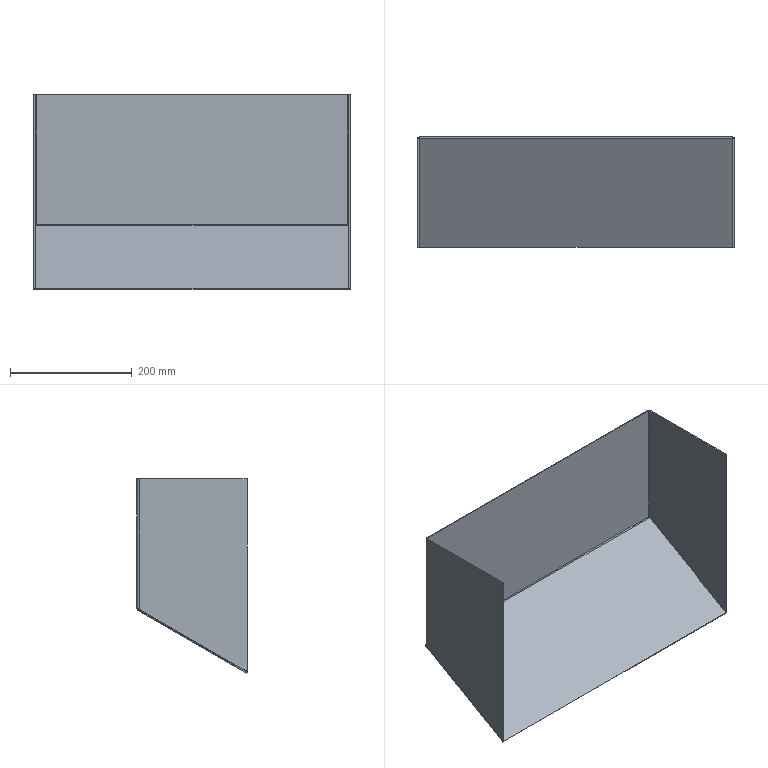Component | SolidWorks | RearLeftSidePlateAssembly-2_RearLeftSidePlateAirInletBaffle-3 | 1 solid | 32 faces | box 520 x 181 x 320 mm | volume 628304 mm3 | plane 24 | cylinder 6 | spline 2 | commonest cylinder face diameters 8 x3 4 x3 | material Plain Carbon Steel
STEP:
#1=COLOUR_RGB('',0.7922,0.8196,0.9333);
#2=FILL_AREA_STYLE_COLOUR('',#1);
#3=FILL_AREA_STYLE('',(#2));
#4=SURFACE_STYLE_FILL_AREA(#3);
#5=SURFACE_SIDE_STYLE('',(#4));
#6=SURFACE_STYLE_USAGE(.BOTH.,#5);
#7=PRESENTATION_STYLE_ASSIGNMENT((#6));
#8=CARTESIAN_POINT('',(98.555,5.691,77.381));
#9=VERTEX_POINT('',#8);
#10=CARTESIAN_POINT('',(98.555,5.691,68.965));
#11=VERTEX_POINT('',#10);
#12=CARTESIAN_POINT('',(98.555,5.691,77.381));
#13=DIRECTION('',(0.,-0.,-1.));
#14=VECTOR('',#13,39.37);
#15=LINE('',#12,#14);
#16=EDGE_CURVE('',#9,#11,#15,.T.);
#17=ORIENTED_EDGE('',*,*,#16,.F.);
#18=CARTESIAN_POINT('',(78.397,5.691,77.381));
#19=VERTEX_POINT('',#18);
#20=CARTESIAN_POINT('',(78.24,5.691,77.381));
#21=DIRECTION('',(1.,0.,-0.));
#22=VECTOR('',#21,39.37);
#23=LINE('',#20,#22);
#24=EDGE_CURVE('',#19,#9,#23,.T.);
#25=ORIENTED_EDGE('',*,*,#24,.F.);
#26=CARTESIAN_POINT('',(78.397,5.691,68.965));
#27=VERTEX_POINT('',#26);
#28=CARTESIAN_POINT('',(78.397,5.691,68.92));
#29=DIRECTION('',(-0.,0.,1.));
#30=VECTOR('',#29,39.37);
#31=LINE('',#28,#30);
#32=EDGE_CURVE('',#27,#19,#31,.T.);
#33=ORIENTED_EDGE('',*,*,#32,.F.);
#34=CARTESIAN_POINT('',(78.24,5.691,68.965));
#35=DIRECTION('',(1.,0.,-0.));
#36=VECTOR('',#35,39.37);
#37=LINE('',#34,#36);
#38=EDGE_CURVE('',#27,#11,#37,.T.);
#39=ORIENTED_EDGE('',*,*,#38,.T.);
#40=EDGE_LOOP('',(#17,#25,#33,#39));
#41=FACE_OUTER_BOUND('',#40,.T.);
#42=CARTESIAN_POINT('',(78.24,5.691,68.874));
#43=DIRECTION('',(-0.,1.,-0.));
#44=DIRECTION('',(-1.,-0.,0.));
#45=AXIS2_PLACEMENT_3D('',#42,#43,#44);
#46=PLANE('',#45);
#47=ADVANCED_FACE('',(#41),#46,.F.);
#48=CARTESIAN_POINT('',(78.397,5.77,77.381));
#49=VERTEX_POINT('',#48);
#50=CARTESIAN_POINT('',(98.555,5.77,77.381));
#51=VERTEX_POINT('',#50);
#52=CARTESIAN_POINT('',(78.24,5.77,77.381));
#53=DIRECTION('',(1.,0.,-0.));
#54=VECTOR('',#53,39.37);
#55=LINE('',#52,#54);
#56=EDGE_CURVE('',#49,#51,#55,.T.);
#57=ORIENTED_EDGE('',*,*,#56,.T.);
#58=CARTESIAN_POINT('',(98.555,5.77,68.965));
#59=VERTEX_POINT('',#58);
#60=CARTESIAN_POINT('',(98.555,5.77,77.381));
#61=DIRECTION('',(0.,-0.,-1.));
#62=VECTOR('',#61,39.37);
#63=LINE('',#60,#62);
#64=EDGE_CURVE('',#51,#59,#63,.T.);
#65=ORIENTED_EDGE('',*,*,#64,.T.);
#66=CARTESIAN_POINT('',(78.397,5.77,68.965));
#67=VERTEX_POINT('',#66);
#68=CARTESIAN_POINT('',(78.24,5.77,68.965));
#69=DIRECTION('',(1.,0.,-0.));
#70=VECTOR('',#69,39.37);
#71=LINE('',#68,#70);
#72=EDGE_CURVE('',#67,#59,#71,.T.);
#73=ORIENTED_EDGE('',*,*,#72,.F.);
#74=CARTESIAN_POINT('',(78.397,5.77,68.92));
#75=DIRECTION('',(-0.,0.,1.));
#76=VECTOR('',#75,39.37);
#77=LINE('',#74,#76);
#78=EDGE_CURVE('',#67,#49,#77,.T.);
#79=ORIENTED_EDGE('',*,*,#78,.T.);
#80=EDGE_LOOP('',(#57,#65,#73,#79));
#81=FACE_OUTER_BOUND('',#80,.T.);
#82=CARTESIAN_POINT('',(78.24,5.77,68.874));
#83=DIRECTION('',(-0.,1.,-0.));
#84=DIRECTION('',(-1.,-0.,0.));
#85=AXIS2_PLACEMENT_3D('',#82,#83,#84);
#86=PLANE('',#85);
#87=ADVANCED_FACE('',(#81),#86,.T.);
#88=ORIENTED_EDGE('',*,*,#24,.T.);
#89=CARTESIAN_POINT('',(98.555,5.691,77.381));
#90=DIRECTION('',(-0.,1.,-0.));
#91=VECTOR('',#90,39.37);
#92=LINE('',#89,#91);
#93=EDGE_CURVE('',#9,#51,#92,.T.);
#94=ORIENTED_EDGE('',*,*,#93,.T.);
#95=ORIENTED_EDGE('',*,*,#56,.F.);
#96=CARTESIAN_POINT('',(78.397,5.691,77.381));
#97=DIRECTION('',(-0.,1.,-0.));
#98=VECTOR('',#97,39.37);
#99=LINE('',#96,#98);
#100=EDGE_CURVE('',#19,#49,#99,.T.);
#101=ORIENTED_EDGE('',*,*,#100,.F.);
#102=EDGE_LOOP('',(#88,#94,#95,#101));
#103=FACE_OUTER_BOUND('',#102,.T.);
#104=CARTESIAN_POINT('',(78.24,5.77,77.381));
#105=DIRECTION('',(0.,0.,1.));
#106=DIRECTION('',(-1.,-0.,0.));
#107=AXIS2_PLACEMENT_3D('',#104,#105,#106);
#108=PLANE('',#107);
#109=ADVANCED_FACE('',(#103),#108,.T.);
#110=CARTESIAN_POINT('',(78.24,5.77,68.965));
#111=VERTEX_POINT('',#110);
#112=CARTESIAN_POINT('',(78.24,5.691,68.965));
#113=VERTEX_POINT('',#112);
#114=CARTESIAN_POINT('',(78.24,5.77,68.965));
#115=DIRECTION('',(0.,-1.,0.));
#116=VECTOR('',#115,39.37);
#117=LINE('',#114,#116);
#118=EDGE_CURVE('',#111,#113,#117,.T.);
#119=ORIENTED_EDGE('',*,*,#118,.F.);
#120=CARTESIAN_POINT('',(78.24,5.691,68.829));
#121=VERTEX_POINT('',#120);
#122=CARTESIAN_POINT('',(78.24,5.612,68.965));
#123=DIRECTION('',(1.,0.,-0.));
#124=DIRECTION('',(0.,-1.,0.));
#125=AXIS2_PLACEMENT_3D('',#122,#123,#124);
#126=CIRCLE('',#125,0.1575);
#127=EDGE_CURVE('',#121,#111,#126,.T.);
#128=ORIENTED_EDGE('',*,*,#127,.F.);
#129=CARTESIAN_POINT('',(78.24,5.652,68.897));
#130=VERTEX_POINT('',#129);
#131=CARTESIAN_POINT('',(78.24,5.652,68.897));
#132=DIRECTION('',(-0.,0.5,-0.866));
#133=VECTOR('',#132,39.37);
#134=LINE('',#131,#133);
#135=EDGE_CURVE('',#130,#121,#134,.T.);
#136=ORIENTED_EDGE('',*,*,#135,.F.);
#137=CARTESIAN_POINT('',(78.24,5.612,68.965));
#138=DIRECTION('',(1.,0.,-0.));
#139=DIRECTION('',(0.,-1.,0.));
#140=AXIS2_PLACEMENT_3D('',#137,#138,#139);
#141=CIRCLE('',#140,0.07874);
#142=EDGE_CURVE('',#130,#113,#141,.T.);
#143=ORIENTED_EDGE('',*,*,#142,.T.);
#144=EDGE_LOOP('',(#119,#128,#136,#143));
#145=FACE_OUTER_BOUND('',#144,.T.);
#146=CARTESIAN_POINT('',(78.24,5.77,68.965));
#147=DIRECTION('',(-1.,-0.,0.));
#148=DIRECTION('',(0.,-1.,0.));
#149=AXIS2_PLACEMENT_3D('',#146,#147,#148);
#150=PLANE('',#149);
#151=ADVANCED_FACE('',(#145),#150,.T.);
#152=CARTESIAN_POINT('',(98.712,5.691,68.829));
#153=VERTEX_POINT('',#152);
#154=CARTESIAN_POINT('',(98.712,5.652,68.897));
#155=VERTEX_POINT('',#154);
#156=CARTESIAN_POINT('',(98.712,5.691,68.829));
#157=DIRECTION('',(0.,-0.5,0.866));
#158=VECTOR('',#157,39.37);
#159=LINE('',#156,#158);
#160=EDGE_CURVE('',#153,#155,#159,.T.);
#161=ORIENTED_EDGE('',*,*,#160,.F.);
#162=CARTESIAN_POINT('',(98.712,5.77,68.965));
#163=VERTEX_POINT('',#162);
#164=CARTESIAN_POINT('',(98.712,5.612,68.965));
#165=DIRECTION('',(1.,0.,-0.));
#166=DIRECTION('',(0.,-1.,0.));
#167=AXIS2_PLACEMENT_3D('',#164,#165,#166);
#168=CIRCLE('',#167,0.1575);
#169=EDGE_CURVE('',#153,#163,#168,.T.);
#170=ORIENTED_EDGE('',*,*,#169,.T.);
#171=CARTESIAN_POINT('',(98.712,5.691,68.965));
#172=VERTEX_POINT('',#171);
#173=CARTESIAN_POINT('',(98.712,5.691,68.965));
#174=DIRECTION('',(-0.,1.,-0.));
#175=VECTOR('',#174,39.37);
#176=LINE('',#173,#175);
#177=EDGE_CURVE('',#172,#163,#176,.T.);
#178=ORIENTED_EDGE('',*,*,#177,.F.);
#179=CARTESIAN_POINT('',(98.712,5.612,68.965));
#180=DIRECTION('',(1.,0.,-0.));
#181=DIRECTION('',(0.,-1.,0.));
#182=AXIS2_PLACEMENT_3D('',#179,#180,#181);
#183=CIRCLE('',#182,0.07874);
#184=EDGE_CURVE('',#155,#172,#183,.T.);
#185=ORIENTED_EDGE('',*,*,#184,.F.);
#186=EDGE_LOOP('',(#161,#170,#178,#185));
#187=FACE_OUTER_BOUND('',#186,.T.);
#188=CARTESIAN_POINT('',(98.712,5.691,68.829));
#189=DIRECTION('',(1.,0.,-0.));
#190=DIRECTION('',(-0.,1.,-0.));
#191=AXIS2_PLACEMENT_3D('',#188,#189,#190);
#192=PLANE('',#191);
#193=ADVANCED_FACE('',(#187),#192,.T.);
#194=CARTESIAN_POINT('',(98.712,-1.317,64.783));
#195=VERTEX_POINT('',#194);
#196=CARTESIAN_POINT('',(98.712,5.77,68.874));
#197=DIRECTION('',(-0.,0.866,0.5));
#198=VECTOR('',#197,39.37);
#199=LINE('',#196,#198);
#200=EDGE_CURVE('',#195,#153,#199,.T.);
#201=ORIENTED_EDGE('',*,*,#200,.T.);
#202=ORIENTED_EDGE('',*,*,#160,.T.);
#203=CARTESIAN_POINT('',(98.712,-1.356,64.851));
#204=VERTEX_POINT('',#203);
#205=CARTESIAN_POINT('',(98.712,5.73,68.942));
#206=DIRECTION('',(-0.,0.866,0.5));
#207=VECTOR('',#206,39.37);
#208=LINE('',#205,#207);
#209=EDGE_CURVE('',#204,#155,#208,.T.);
#210=ORIENTED_EDGE('',*,*,#209,.F.);
#211=CARTESIAN_POINT('',(98.712,-1.356,64.851));
#212=DIRECTION('',(-0.,0.5,-0.866));
#213=VECTOR('',#212,39.37);
#214=LINE('',#211,#213);
#215=EDGE_CURVE('',#204,#195,#214,.T.);
#216=ORIENTED_EDGE('',*,*,#215,.T.);
#217=EDGE_LOOP('',(#201,#202,#210,#216));
#218=FACE_OUTER_BOUND('',#217,.T.);
#219=CARTESIAN_POINT('',(98.712,5.691,68.965));
#220=DIRECTION('',(1.,0.,-0.));
#221=DIRECTION('',(-0.,1.,-0.));
#222=AXIS2_PLACEMENT_3D('',#219,#220,#221);
#223=PLANE('',#222);
#224=ADVANCED_FACE('',(#218),#223,.T.);
#225=ORIENTED_EDGE('',*,*,#169,.F.);
#226=CARTESIAN_POINT('',(78.24,5.691,68.829));
#227=DIRECTION('',(1.,0.,-0.));
#228=VECTOR('',#227,39.37);
#229=LINE('',#226,#228);
#230=EDGE_CURVE('',#121,#153,#229,.T.);
#231=ORIENTED_EDGE('',*,*,#230,.F.);
#232=ORIENTED_EDGE('',*,*,#127,.T.);
#233=CARTESIAN_POINT('',(78.24,5.77,68.965));
#234=DIRECTION('',(1.,0.,-0.));
#235=VECTOR('',#234,39.37);
#236=LINE('',#233,#235);
#237=EDGE_CURVE('',#111,#67,#236,.T.);
#238=ORIENTED_EDGE('',*,*,#237,.T.);
#239=ORIENTED_EDGE('',*,*,#72,.T.);
#240=CARTESIAN_POINT('',(78.24,5.77,68.965));
#241=DIRECTION('',(1.,0.,-0.));
#242=VECTOR('',#241,39.37);
#243=LINE('',#240,#242);
#244=EDGE_CURVE('',#59,#163,#243,.T.);
#245=ORIENTED_EDGE('',*,*,#244,.T.);
#246=EDGE_LOOP('',(#225,#231,#232,#238,#239,#245));
#247=FACE_OUTER_BOUND('',#246,.T.);
#248=CARTESIAN_POINT('',(78.24,5.612,68.965));
#249=DIRECTION('',(1.,0.,-0.));
#250=DIRECTION('',(0.,1.,0.));
#251=AXIS2_PLACEMENT_3D('',#248,#249,#250);
#252=CYLINDRICAL_SURFACE('',#251,0.1575);
#253=ADVANCED_FACE('',(#247),#252,.T.);
#254=ORIENTED_EDGE('',*,*,#200,.F.);
#255=CARTESIAN_POINT('',(78.24,-1.317,64.783));
#256=VERTEX_POINT('',#255);
#257=CARTESIAN_POINT('',(78.24,-1.317,64.783));
#258=DIRECTION('',(1.,0.,-0.));
#259=VECTOR('',#258,39.37);
#260=LINE('',#257,#259);
#261=EDGE_CURVE('',#256,#195,#260,.T.);
#262=ORIENTED_EDGE('',*,*,#261,.F.);
#263=CARTESIAN_POINT('',(78.24,5.77,68.874));
#264=DIRECTION('',(-0.,0.866,0.5));
#265=VECTOR('',#264,39.37);
#266=LINE('',#263,#265);
#267=EDGE_CURVE('',#256,#121,#266,.T.);
#268=ORIENTED_EDGE('',*,*,#267,.T.);
#269=ORIENTED_EDGE('',*,*,#230,.T.);
#270=EDGE_LOOP('',(#254,#262,#268,#269));
#271=FACE_OUTER_BOUND('',#270,.T.);
#272=CARTESIAN_POINT('',(78.24,5.77,68.874));
#273=DIRECTION('',(-0.,0.5,-0.866));
#274=DIRECTION('',(0.,-0.866,-0.5));
#275=AXIS2_PLACEMENT_3D('',#272,#273,#274);
#276=PLANE('',#275);
#277=ADVANCED_FACE('',(#271),#276,.T.);
#278=ORIENTED_EDGE('',*,*,#215,.F.);
#279=CARTESIAN_POINT('',(78.24,-1.356,64.851));
#280=VERTEX_POINT('',#279);
#281=CARTESIAN_POINT('',(78.24,-1.356,64.851));
#282=DIRECTION('',(1.,0.,-0.));
#283=VECTOR('',#282,39.37);
#284=LINE('',#281,#283);
#285=EDGE_CURVE('',#280,#204,#284,.T.);
#286=ORIENTED_EDGE('',*,*,#285,.F.);
#287=CARTESIAN_POINT('',(78.24,-1.356,64.851));
#288=DIRECTION('',(-0.,0.5,-0.866));
#289=VECTOR('',#288,39.37);
#290=LINE('',#287,#289);
#291=EDGE_CURVE('',#280,#256,#290,.T.);
#292=ORIENTED_EDGE('',*,*,#291,.T.);
#293=ORIENTED_EDGE('',*,*,#261,.T.);
#294=EDGE_LOOP('',(#278,#286,#292,#293));
#295=FACE_OUTER_BOUND('',#294,.T.);
#296=CARTESIAN_POINT('',(78.24,-1.356,64.851));
#297=DIRECTION('',(0.,-0.866,-0.5));
#298=DIRECTION('',(0.,-0.5,0.866));
#299=AXIS2_PLACEMENT_3D('',#296,#297,#298);
#300=PLANE('',#299);
#301=ADVANCED_FACE('',(#295),#300,.T.);
#302=ORIENTED_EDGE('',*,*,#209,.T.);
#303=CARTESIAN_POINT('',(78.24,5.652,68.897));
#304=DIRECTION('',(1.,0.,-0.));
#305=VECTOR('',#304,39.37);
#306=LINE('',#303,#305);
#307=EDGE_CURVE('',#130,#155,#306,.T.);
#308=ORIENTED_EDGE('',*,*,#307,.F.);
#309=CARTESIAN_POINT('',(78.24,5.73,68.942));
#310=DIRECTION('',(-0.,0.866,0.5));
#311=VECTOR('',#310,39.37);
#312=LINE('',#309,#311);
#313=EDGE_CURVE('',#280,#130,#312,.T.);
#314=ORIENTED_EDGE('',*,*,#313,.F.);
#315=ORIENTED_EDGE('',*,*,#285,.T.);
#316=EDGE_LOOP('',(#302,#308,#314,#315));
#317=FACE_OUTER_BOUND('',#316,.T.);
#318=CARTESIAN_POINT('',(78.24,5.73,68.942));
#319=DIRECTION('',(-0.,0.5,-0.866));
#320=DIRECTION('',(0.,-0.866,-0.5));
#321=AXIS2_PLACEMENT_3D('',#318,#319,#320);
#322=PLANE('',#321);
#323=ADVANCED_FACE('',(#317),#322,.F.);
#324=ORIENTED_EDGE('',*,*,#184,.T.);
#325=CARTESIAN_POINT('',(98.555,5.691,68.965));
#326=DIRECTION('',(1.,0.,0.));
#327=VECTOR('',#326,39.37);
#328=LINE('',#325,#327);
#329=EDGE_CURVE('',#11,#172,#328,.T.);
#330=ORIENTED_EDGE('',*,*,#329,.F.);
#331=ORIENTED_EDGE('',*,*,#38,.F.);
#332=CARTESIAN_POINT('',(78.24,5.691,68.965));
#333=DIRECTION('',(1.,0.,-0.));
#334=VECTOR('',#333,39.37);
#335=LINE('',#332,#334);
#336=EDGE_CURVE('',#113,#27,#335,.T.);
#337=ORIENTED_EDGE('',*,*,#336,.F.);
#338=ORIENTED_EDGE('',*,*,#142,.F.);
#339=ORIENTED_EDGE('',*,*,#307,.T.);
#340=EDGE_LOOP('',(#324,#330,#331,#337,#338,#339));
#341=FACE_OUTER_BOUND('',#340,.T.);
#342=CARTESIAN_POINT('',(78.24,5.612,68.965));
#343=DIRECTION('',(1.,0.,-0.));
#344=DIRECTION('',(0.,1.,0.));
#345=AXIS2_PLACEMENT_3D('',#342,#343,#344);
#346=CYLINDRICAL_SURFACE('',#345,0.07874);
#347=ADVANCED_FACE('',(#341),#346,.F.);
#348=ORIENTED_EDGE('',*,*,#313,.T.);
#349=ORIENTED_EDGE('',*,*,#135,.T.);
#350=ORIENTED_EDGE('',*,*,#267,.F.);
#351=ORIENTED_EDGE('',*,*,#291,.F.);
#352=EDGE_LOOP('',(#348,#349,#350,#351));
#353=FACE_OUTER_BOUND('',#352,.T.);
#354=CARTESIAN_POINT('',(78.24,5.612,68.965));
#355=DIRECTION('',(-1.,-0.,0.));
#356=DIRECTION('',(0.,-1.,0.));
#357=AXIS2_PLACEMENT_3D('',#354,#355,#356);
#358=PLANE('',#357);
#359=ADVANCED_FACE('',(#353),#358,.T.);
#360=ORIENTED_EDGE('',*,*,#237,.F.);
#361=ORIENTED_EDGE('',*,*,#118,.T.);
#362=ORIENTED_EDGE('',*,*,#336,.T.);
#363=CARTESIAN_POINT('',(78.397,5.691,68.965));
#364=DIRECTION('',(-0.,1.,-0.));
#365=VECTOR('',#364,39.37);
#366=LINE('',#363,#365);
#367=EDGE_CURVE('',#27,#67,#366,.T.);
#368=ORIENTED_EDGE('',*,*,#367,.T.);
#369=EDGE_LOOP('',(#360,#361,#362,#368));
#370=FACE_OUTER_BOUND('',#369,.T.);
#371=CARTESIAN_POINT('',(78.24,5.691,68.965));
#372=DIRECTION('',(0.,0.,1.));
#373=DIRECTION('',(-1.,-0.,0.));
#374=AXIS2_PLACEMENT_3D('',#371,#372,#373);
#375=PLANE('',#374);
#376=ADVANCED_FACE('',(#370),#375,.T.);
#377=CARTESIAN_POINT('',(78.318,5.612,77.381));
#378=VERTEX_POINT('',#377);
#379=CARTESIAN_POINT('',(78.24,5.612,77.381));
#380=VERTEX_POINT('',#379);
#381=CARTESIAN_POINT('',(78.24,5.612,77.381));
#382=DIRECTION('',(-1.,-0.,0.));
#383=VECTOR('',#382,39.37);
#384=LINE('',#381,#383);
#385=EDGE_CURVE('',#378,#380,#384,.T.);
#386=ORIENTED_EDGE('',*,*,#385,.F.);
#387=CARTESIAN_POINT('',(78.397,5.612,77.381));
#388=DIRECTION('',(-0.,0.,1.));
#389=DIRECTION('',(1.,0.,0.));
#390=AXIS2_PLACEMENT_3D('',#387,#388,#389);
#391=CIRCLE('',#390,0.07874);
#392=EDGE_CURVE('',#19,#378,#391,.T.);
#393=ORIENTED_EDGE('',*,*,#392,.F.);
#394=ORIENTED_EDGE('',*,*,#100,.T.);
#395=CARTESIAN_POINT('',(78.397,5.612,77.381));
#396=DIRECTION('',(-0.,0.,1.));
#397=DIRECTION('',(1.,0.,0.));
#398=AXIS2_PLACEMENT_3D('',#395,#396,#397);
#399=CIRCLE('',#398,0.1575);
#400=EDGE_CURVE('',#49,#380,#399,.T.);
#401=ORIENTED_EDGE('',*,*,#400,.T.);
#402=EDGE_LOOP('',(#386,#393,#394,#401));
#403=FACE_OUTER_BOUND('',#402,.T.);
#404=CARTESIAN_POINT('',(78.397,5.612,77.381));
#405=DIRECTION('',(0.,0.,1.));
#406=DIRECTION('',(-1.,-0.,0.));
#407=AXIS2_PLACEMENT_3D('',#404,#405,#406);
#408=PLANE('',#407);
#409=ADVANCED_FACE('',(#403),#408,.T.);
#410=CARTESIAN_POINT('',(78.318,5.612,68.92));
#411=VERTEX_POINT('',#410);
#412=CARTESIAN_POINT('',(78.318,5.612,68.92));
#413=CARTESIAN_POINT('',(78.318,5.617,68.921));
#414=CARTESIAN_POINT('',(78.319,5.622,68.923));
#415=CARTESIAN_POINT('',(78.321,5.633,68.927));
#416=CARTESIAN_POINT('',(78.322,5.638,68.929));
#417=CARTESIAN_POINT('',(78.326,5.647,68.933));
#418=CARTESIAN_POINT('',(78.329,5.652,68.935));
#419=CARTESIAN_POINT('',(78.334,5.66,68.938));
#420=CARTESIAN_POINT('',(78.338,5.664,68.94));
#421=CARTESIAN_POINT('',(78.345,5.671,68.944));
#422=CARTESIAN_POINT('',(78.349,5.675,68.946));
#423=CARTESIAN_POINT('',(78.358,5.68,68.95));
#424=CARTESIAN_POINT('',(78.362,5.683,68.952));
#425=CARTESIAN_POINT('',(78.372,5.687,68.956));
#426=CARTESIAN_POINT('',(78.377,5.688,68.957));
#427=CARTESIAN_POINT('',(78.387,5.69,68.961));
#428=CARTESIAN_POINT('',(78.392,5.691,68.963));
#429=CARTESIAN_POINT('',(78.397,5.691,68.965));
#430=B_SPLINE_CURVE_WITH_KNOTS('',3,(#412,#413,#414,#415,#416,#417,#418,#419,#420,#421,#422,#423,#424,#425,#426,#427,#428,#429),.UNSPECIFIED.,.F.,.F.,(4,2,2,2,2,2,2,2,4),(0.,0.0004161,0.0008322,0.001248,0.001664,0.002081,0.002497,0.002913,0.003329),.UNSPECIFIED.);
#431=EDGE_CURVE('',#411,#27,#430,.T.);
#432=ORIENTED_EDGE('',*,*,#431,.F.);
#433=CARTESIAN_POINT('',(78.24,5.612,68.92));
#434=VERTEX_POINT('',#433);
#435=CARTESIAN_POINT('',(78.318,5.612,68.92));
#436=DIRECTION('',(-1.,-0.,-0.));
#437=VECTOR('',#436,39.37);
#438=LINE('',#435,#437);
#439=EDGE_CURVE('',#411,#434,#438,.T.);
#440=ORIENTED_EDGE('',*,*,#439,.T.);
#441=CARTESIAN_POINT('',(78.24,5.612,68.92));
#442=CARTESIAN_POINT('',(78.24,5.623,68.921));
#443=CARTESIAN_POINT('',(78.241,5.633,68.923));
#444=CARTESIAN_POINT('',(78.245,5.653,68.927));
#445=CARTESIAN_POINT('',(78.248,5.663,68.929));
#446=CARTESIAN_POINT('',(78.256,5.682,68.933));
#447=CARTESIAN_POINT('',(78.26,5.691,68.935));
#448=CARTESIAN_POINT('',(78.272,5.708,68.938));
#449=CARTESIAN_POINT('',(78.278,5.716,68.94));
#450=CARTESIAN_POINT('',(78.293,5.731,68.944));
#451=CARTESIAN_POINT('',(78.301,5.737,68.946));
#452=CARTESIAN_POINT('',(78.318,5.749,68.95));
#453=CARTESIAN_POINT('',(78.327,5.754,68.952));
#454=CARTESIAN_POINT('',(78.356,5.765,68.957));
#455=CARTESIAN_POINT('',(78.376,5.77,68.961));
#456=CARTESIAN_POINT('',(78.397,5.77,68.965));
#457=B_SPLINE_CURVE_WITH_KNOTS('',3,(#441,#442,#443,#444,#445,#446,#447,#448,#449,#450,#451,#452,#453,#454,#455,#456),.UNSPECIFIED.,.F.,.F.,(4,2,2,2,2,2,2,4),(0.,0.0007941,0.001588,0.002382,0.003177,0.003971,0.004765,0.006353),.UNSPECIFIED.);
#458=EDGE_CURVE('',#434,#67,#457,.T.);
#459=ORIENTED_EDGE('',*,*,#458,.T.);
#460=ORIENTED_EDGE('',*,*,#367,.F.);
#461=EDGE_LOOP('',(#432,#440,#459,#460));
#462=FACE_OUTER_BOUND('',#461,.T.);
#463=CARTESIAN_POINT('',(78.239,5.612,68.92));
#464=CARTESIAN_POINT('',(78.239,5.633,68.923));
#465=CARTESIAN_POINT('',(78.243,5.654,68.927));
#466=CARTESIAN_POINT('',(78.259,5.692,68.935));
#467=CARTESIAN_POINT('',(78.271,5.709,68.938));
#468=CARTESIAN_POINT('',(78.3,5.739,68.946));
#469=CARTESIAN_POINT('',(78.317,5.75,68.95));
#470=CARTESIAN_POINT('',(78.356,5.766,68.957));
#471=CARTESIAN_POINT('',(78.376,5.77,68.961));
#472=CARTESIAN_POINT('',(78.397,5.77,68.965));
#473=CARTESIAN_POINT('',(78.24,5.612,68.92));
#474=CARTESIAN_POINT('',(78.24,5.633,68.923));
#475=CARTESIAN_POINT('',(78.244,5.653,68.927));
#476=CARTESIAN_POINT('',(78.26,5.691,68.935));
#477=CARTESIAN_POINT('',(78.271,5.709,68.938));
#478=CARTESIAN_POINT('',(78.3,5.738,68.946));
#479=CARTESIAN_POINT('',(78.318,5.75,68.95));
#480=CARTESIAN_POINT('',(78.356,5.766,68.957));
#481=CARTESIAN_POINT('',(78.377,5.77,68.961));
#482=CARTESIAN_POINT('',(78.397,5.77,68.965));
#483=CARTESIAN_POINT('',(78.318,5.612,68.92));
#484=CARTESIAN_POINT('',(78.318,5.622,68.923));
#485=CARTESIAN_POINT('',(78.32,5.633,68.927));
#486=CARTESIAN_POINT('',(78.328,5.652,68.935));
#487=CARTESIAN_POINT('',(78.334,5.661,68.938));
#488=CARTESIAN_POINT('',(78.349,5.675,68.946));
#489=CARTESIAN_POINT('',(78.357,5.681,68.95));
#490=CARTESIAN_POINT('',(78.377,5.689,68.957));
#491=CARTESIAN_POINT('',(78.387,5.691,68.961));
#492=CARTESIAN_POINT('',(78.397,5.691,68.965));
#493=CARTESIAN_POINT('',(78.319,5.612,68.92));
#494=CARTESIAN_POINT('',(78.319,5.622,68.923));
#495=CARTESIAN_POINT('',(78.321,5.633,68.927));
#496=CARTESIAN_POINT('',(78.329,5.651,68.935));
#497=CARTESIAN_POINT('',(78.335,5.66,68.938));
#498=CARTESIAN_POINT('',(78.349,5.674,68.946));
#499=CARTESIAN_POINT('',(78.358,5.68,68.95));
#500=CARTESIAN_POINT('',(78.377,5.688,68.957));
#501=CARTESIAN_POINT('',(78.387,5.69,68.961));
#502=CARTESIAN_POINT('',(78.397,5.69,68.965));
#503=B_SPLINE_SURFACE_WITH_KNOTS('',1,3,((#463,#464,#465,#466,#467,#468,#469,#470,#471,#472),(#473,#474,#475,#476,#477,#478,#479,#480,#481,#482),(#483,#484,#485,#486,#487,#488,#489,#490,#491,#492),(#493,#494,#495,#496,#497,#498,#499,#500,#501,#502)),.UNSPECIFIED.,.F.,.F.,.F.,(2,1,1,2),(4,2,2,2,4),(-0.01,0.,1.,1.01),(0.,0.25,0.5,0.75,1.),.UNSPECIFIED.);
#504=ADVANCED_FACE('',(#462),#503,.F.);
#505=ORIENTED_EDGE('',*,*,#78,.F.);
#506=ORIENTED_EDGE('',*,*,#458,.F.);
#507=CARTESIAN_POINT('',(78.24,5.612,77.381));
#508=DIRECTION('',(0.,0.,1.));
#509=VECTOR('',#508,39.37);
#510=LINE('',#507,#509);
#511=EDGE_CURVE('',#434,#380,#510,.T.);
#512=ORIENTED_EDGE('',*,*,#511,.T.);
#513=ORIENTED_EDGE('',*,*,#400,.F.);
#514=EDGE_LOOP('',(#505,#506,#512,#513));
#515=FACE_OUTER_BOUND('',#514,.T.);
#516=CARTESIAN_POINT('',(78.397,5.612,68.92));
#517=DIRECTION('',(0.,-0.,-1.));
#518=DIRECTION('',(-1.,0.,0.));
#519=AXIS2_PLACEMENT_3D('',#516,#517,#518);
#520=CYLINDRICAL_SURFACE('',#519,0.1575);
#521=ADVANCED_FACE('',(#515),#520,.T.);
#522=ORIENTED_EDGE('',*,*,#32,.T.);
#523=ORIENTED_EDGE('',*,*,#392,.T.);
#524=CARTESIAN_POINT('',(78.318,5.612,77.381));
#525=DIRECTION('',(-0.,-0.,-1.));
#526=VECTOR('',#525,39.37);
#527=LINE('',#524,#526);
#528=EDGE_CURVE('',#378,#411,#527,.T.);
#529=ORIENTED_EDGE('',*,*,#528,.T.);
#530=ORIENTED_EDGE('',*,*,#431,.T.);
#531=EDGE_LOOP('',(#522,#523,#529,#530));
#532=FACE_OUTER_BOUND('',#531,.T.);
#533=CARTESIAN_POINT('',(78.397,5.612,68.92));
#534=DIRECTION('',(0.,-0.,-1.));
#535=DIRECTION('',(-1.,0.,0.));
#536=AXIS2_PLACEMENT_3D('',#533,#534,#535);
#537=CYLINDRICAL_SURFACE('',#536,0.07874);
#538=ADVANCED_FACE('',(#532),#537,.F.);
#539=ORIENTED_EDGE('',*,*,#439,.F.);
#540=CARTESIAN_POINT('',(78.318,-1.356,64.896));
#541=VERTEX_POINT('',#540);
#542=CARTESIAN_POINT('',(78.318,5.691,68.965));
#543=DIRECTION('',(-0.,-0.866,-0.5));
#544=VECTOR('',#543,39.37);
#545=LINE('',#542,#544);
#546=EDGE_CURVE('',#411,#541,#545,.T.);
#547=ORIENTED_EDGE('',*,*,#546,.T.);
#548=CARTESIAN_POINT('',(78.24,-1.356,64.896));
#549=VERTEX_POINT('',#548);
#550=CARTESIAN_POINT('',(78.24,-1.356,64.896));
#551=DIRECTION('',(1.,0.,0.));
#552=VECTOR('',#551,39.37);
#553=LINE('',#550,#552);
#554=EDGE_CURVE('',#549,#541,#553,.T.);
#555=ORIENTED_EDGE('',*,*,#554,.F.);
#556=CARTESIAN_POINT('',(78.24,5.711,68.976));
#557=DIRECTION('',(-0.,-0.866,-0.5));
#558=VECTOR('',#557,39.37);
#559=LINE('',#556,#558);
#560=EDGE_CURVE('',#434,#549,#559,.T.);
#561=ORIENTED_EDGE('',*,*,#560,.F.);
#562=EDGE_LOOP('',(#539,#547,#555,#561));
#563=FACE_OUTER_BOUND('',#562,.T.);
#564=CARTESIAN_POINT('',(78.24,5.691,68.965));
#565=DIRECTION('',(0.,-0.5,0.866));
#566=DIRECTION('',(-0.,0.866,0.5));
#567=AXIS2_PLACEMENT_3D('',#564,#565,#566);
#568=PLANE('',#567);
#569=ADVANCED_FACE('',(#563),#568,.F.);
#570=ORIENTED_EDGE('',*,*,#385,.T.);
#571=CARTESIAN_POINT('',(78.24,-1.356,77.381));
#572=VERTEX_POINT('',#571);
#573=CARTESIAN_POINT('',(78.24,5.77,77.381));
#574=DIRECTION('',(0.,1.,-0.));
#575=VECTOR('',#574,39.37);
#576=LINE('',#573,#575);
#577=EDGE_CURVE('',#572,#380,#576,.T.);
#578=ORIENTED_EDGE('',*,*,#577,.F.);
#579=CARTESIAN_POINT('',(78.318,-1.356,77.381));
#580=VERTEX_POINT('',#579);
#581=CARTESIAN_POINT('',(78.24,-1.356,77.381));
#582=DIRECTION('',(1.,0.,0.));
#583=VECTOR('',#582,39.37);
#584=LINE('',#581,#583);
#585=EDGE_CURVE('',#572,#580,#584,.T.);
#586=ORIENTED_EDGE('',*,*,#585,.T.);
#587=CARTESIAN_POINT('',(78.318,5.691,77.381));
#588=DIRECTION('',(0.,1.,-0.));
#589=VECTOR('',#588,39.37);
#590=LINE('',#587,#589);
#591=EDGE_CURVE('',#580,#378,#590,.T.);
#592=ORIENTED_EDGE('',*,*,#591,.T.);
#593=EDGE_LOOP('',(#570,#578,#586,#592));
#594=FACE_OUTER_BOUND('',#593,.T.);
#595=CARTESIAN_POINT('',(78.24,5.691,77.381));
#596=DIRECTION('',(-0.,-0.,-1.));
#597=DIRECTION('',(1.,0.,-0.));
#598=AXIS2_PLACEMENT_3D('',#595,#596,#597);
#599=PLANE('',#598);
#600=ADVANCED_FACE('',(#594),#599,.F.);
#601=ORIENTED_EDGE('',*,*,#511,.F.);
#602=ORIENTED_EDGE('',*,*,#560,.T.);
#603=CARTESIAN_POINT('',(78.24,-1.356,68.874));
#604=DIRECTION('',(-0.,0.,1.));
#605=VECTOR('',#604,39.37);
#606=LINE('',#603,#605);
#607=EDGE_CURVE('',#549,#572,#606,.T.);
#608=ORIENTED_EDGE('',*,*,#607,.T.);
#609=ORIENTED_EDGE('',*,*,#577,.T.);
#610=EDGE_LOOP('',(#601,#602,#608,#609));
#611=FACE_OUTER_BOUND('',#610,.T.);
#612=CARTESIAN_POINT('',(78.24,5.77,68.874));
#613=DIRECTION('',(1.,-0.,0.));
#614=DIRECTION('',(0.,1.,-0.));
#615=AXIS2_PLACEMENT_3D('',#612,#613,#614);
#616=PLANE('',#615);
#617=ADVANCED_FACE('',(#611),#616,.F.);
#618=ORIENTED_EDGE('',*,*,#546,.F.);
#619=ORIENTED_EDGE('',*,*,#528,.F.);
#620=ORIENTED_EDGE('',*,*,#591,.F.);
#621=CARTESIAN_POINT('',(78.318,-1.356,77.381));
#622=DIRECTION('',(-0.,0.,1.));
#623=VECTOR('',#622,39.37);
#624=LINE('',#621,#623);
#625=EDGE_CURVE('',#541,#580,#624,.T.);
#626=ORIENTED_EDGE('',*,*,#625,.F.);
#627=EDGE_LOOP('',(#618,#619,#620,#626));
#628=FACE_OUTER_BOUND('',#627,.T.);
#629=CARTESIAN_POINT('',(78.318,5.77,68.874));
#630=DIRECTION('',(1.,-0.,0.));
#631=DIRECTION('',(0.,1.,-0.));
#632=AXIS2_PLACEMENT_3D('',#629,#630,#631);
#633=PLANE('',#632);
#634=ADVANCED_FACE('',(#628),#633,.T.);
#635=ORIENTED_EDGE('',*,*,#625,.T.);
#636=ORIENTED_EDGE('',*,*,#585,.F.);
#637=ORIENTED_EDGE('',*,*,#607,.F.);
#638=ORIENTED_EDGE('',*,*,#554,.T.);
#639=EDGE_LOOP('',(#635,#636,#637,#638));
#640=FACE_OUTER_BOUND('',#639,.T.);
#641=CARTESIAN_POINT('',(78.24,-1.356,77.381));
#642=DIRECTION('',(0.,1.,-0.));
#643=DIRECTION('',(-1.,0.,-0.));
#644=AXIS2_PLACEMENT_3D('',#641,#642,#643);
#645=PLANE('',#644);
#646=ADVANCED_FACE('',(#640),#645,.F.);
#647=ORIENTED_EDGE('',*,*,#244,.F.);
#648=CARTESIAN_POINT('',(98.555,5.691,68.965));
#649=DIRECTION('',(-0.,1.,-0.));
#650=VECTOR('',#649,39.37);
#651=LINE('',#648,#650);
#652=EDGE_CURVE('',#11,#59,#651,.T.);
#653=ORIENTED_EDGE('',*,*,#652,.F.);
#654=ORIENTED_EDGE('',*,*,#329,.T.);
#655=ORIENTED_EDGE('',*,*,#177,.T.);
#656=EDGE_LOOP('',(#647,#653,#654,#655));
#657=FACE_OUTER_BOUND('',#656,.T.);
#658=CARTESIAN_POINT('',(98.555,5.691,68.965));
#659=DIRECTION('',(-0.,-0.,1.));
#660=DIRECTION('',(-1.,-0.,-0.));
#661=AXIS2_PLACEMENT_3D('',#658,#659,#660);
#662=PLANE('',#661);
#663=ADVANCED_FACE('',(#657),#662,.T.);
#664=CARTESIAN_POINT('',(98.633,5.612,68.92));
#665=VERTEX_POINT('',#664);
#666=CARTESIAN_POINT('',(98.712,5.612,68.92));
#667=VERTEX_POINT('',#666);
#668=CARTESIAN_POINT('',(98.712,5.612,68.92));
#669=DIRECTION('',(1.,0.,-0.));
#670=VECTOR('',#669,39.37);
#671=LINE('',#668,#670);
#672=EDGE_CURVE('',#665,#667,#671,.T.);
#673=ORIENTED_EDGE('',*,*,#672,.F.);
#674=CARTESIAN_POINT('',(98.555,5.691,68.965));
#675=CARTESIAN_POINT('',(98.56,5.691,68.963));
#676=CARTESIAN_POINT('',(98.565,5.69,68.961));
#677=CARTESIAN_POINT('',(98.575,5.688,68.957));
#678=CARTESIAN_POINT('',(98.58,5.687,68.956));
#679=CARTESIAN_POINT('',(98.59,5.683,68.952));
#680=CARTESIAN_POINT('',(98.594,5.681,68.95));
#681=CARTESIAN_POINT('',(98.603,5.675,68.946));
#682=CARTESIAN_POINT('',(98.607,5.671,68.944));
#683=CARTESIAN_POINT('',(98.614,5.664,68.94));
#684=CARTESIAN_POINT('',(98.617,5.66,68.939));
#685=CARTESIAN_POINT('',(98.623,5.652,68.935));
#686=CARTESIAN_POINT('',(98.625,5.647,68.933));
#687=CARTESIAN_POINT('',(98.629,5.638,68.929));
#688=CARTESIAN_POINT('',(98.631,5.633,68.927));
#689=CARTESIAN_POINT('',(98.633,5.623,68.923));
#690=CARTESIAN_POINT('',(98.633,5.617,68.921));
#691=CARTESIAN_POINT('',(98.633,5.612,68.92));
#692=B_SPLINE_CURVE_WITH_KNOTS('',3,(#674,#675,#676,#677,#678,#679,#680,#681,#682,#683,#684,#685,#686,#687,#688,#689,#690,#691),.UNSPECIFIED.,.F.,.F.,(4,2,2,2,2,2,2,2,4),(0.,0.0004161,0.0008322,0.001248,0.001664,0.002081,0.002497,0.002913,0.003329),.UNSPECIFIED.);
#693=EDGE_CURVE('',#11,#665,#692,.T.);
#694=ORIENTED_EDGE('',*,*,#693,.F.);
#695=ORIENTED_EDGE('',*,*,#652,.T.);
#696=CARTESIAN_POINT('',(98.555,5.77,68.965));
#697=CARTESIAN_POINT('',(98.565,5.77,68.963));
#698=CARTESIAN_POINT('',(98.575,5.769,68.961));
#699=CARTESIAN_POINT('',(98.595,5.765,68.957));
#700=CARTESIAN_POINT('',(98.605,5.762,68.956));
#701=CARTESIAN_POINT('',(98.624,5.754,68.952));
#702=CARTESIAN_POINT('',(98.633,5.749,68.95));
#703=CARTESIAN_POINT('',(98.651,5.737,68.946));
#704=CARTESIAN_POINT('',(98.659,5.731,68.944));
#705=CARTESIAN_POINT('',(98.673,5.716,68.94));
#706=CARTESIAN_POINT('',(98.68,5.708,68.939));
#707=CARTESIAN_POINT('',(98.691,5.691,68.935));
#708=CARTESIAN_POINT('',(98.696,5.682,68.933));
#709=CARTESIAN_POINT('',(98.708,5.654,68.927));
#710=CARTESIAN_POINT('',(98.712,5.633,68.923));
#711=CARTESIAN_POINT('',(98.712,5.612,68.92));
#712=B_SPLINE_CURVE_WITH_KNOTS('',3,(#696,#697,#698,#699,#700,#701,#702,#703,#704,#705,#706,#707,#708,#709,#710,#711),.UNSPECIFIED.,.F.,.F.,(4,2,2,2,2,2,2,4),(0.,0.0007941,0.001588,0.002382,0.003177,0.003971,0.004765,0.006353),.UNSPECIFIED.);
#713=EDGE_CURVE('',#59,#667,#712,.T.);
#714=ORIENTED_EDGE('',*,*,#713,.T.);
#715=EDGE_LOOP('',(#673,#694,#695,#714));
#716=FACE_OUTER_BOUND('',#715,.T.);
#717=CARTESIAN_POINT('',(98.555,5.77,68.965));
#718=CARTESIAN_POINT('',(98.575,5.77,68.961));
#719=CARTESIAN_POINT('',(98.596,5.766,68.957));
#720=CARTESIAN_POINT('',(98.634,5.75,68.95));
#721=CARTESIAN_POINT('',(98.652,5.739,68.946));
#722=CARTESIAN_POINT('',(98.681,5.709,68.938));
#723=CARTESIAN_POINT('',(98.693,5.692,68.935));
#724=CARTESIAN_POINT('',(98.709,5.654,68.927));
#725=CARTESIAN_POINT('',(98.713,5.633,68.923));
#726=CARTESIAN_POINT('',(98.713,5.612,68.92));
#727=CARTESIAN_POINT('',(98.555,5.77,68.965));
#728=CARTESIAN_POINT('',(98.575,5.77,68.961));
#729=CARTESIAN_POINT('',(98.596,5.766,68.957));
#730=CARTESIAN_POINT('',(98.634,5.75,68.95));
#731=CARTESIAN_POINT('',(98.651,5.738,68.946));
#732=CARTESIAN_POINT('',(98.681,5.709,68.938));
#733=CARTESIAN_POINT('',(98.692,5.691,68.935));
#734=CARTESIAN_POINT('',(98.708,5.653,68.927));
#735=CARTESIAN_POINT('',(98.712,5.633,68.923));
#736=CARTESIAN_POINT('',(98.712,5.612,68.92));
#737=CARTESIAN_POINT('',(98.555,5.691,68.965));
#738=CARTESIAN_POINT('',(98.565,5.691,68.961));
#739=CARTESIAN_POINT('',(98.575,5.689,68.957));
#740=CARTESIAN_POINT('',(98.594,5.681,68.95));
#741=CARTESIAN_POINT('',(98.603,5.675,68.946));
#742=CARTESIAN_POINT('',(98.618,5.661,68.938));
#743=CARTESIAN_POINT('',(98.623,5.652,68.935));
#744=CARTESIAN_POINT('',(98.631,5.633,68.927));
#745=CARTESIAN_POINT('',(98.633,5.622,68.923));
#746=CARTESIAN_POINT('',(98.633,5.612,68.92));
#747=CARTESIAN_POINT('',(98.555,5.69,68.965));
#748=CARTESIAN_POINT('',(98.565,5.69,68.961));
#749=CARTESIAN_POINT('',(98.575,5.688,68.957));
#750=CARTESIAN_POINT('',(98.594,5.68,68.95));
#751=CARTESIAN_POINT('',(98.603,5.674,68.946));
#752=CARTESIAN_POINT('',(98.617,5.66,68.938));
#753=CARTESIAN_POINT('',(98.623,5.651,68.935));
#754=CARTESIAN_POINT('',(98.631,5.633,68.927));
#755=CARTESIAN_POINT('',(98.633,5.622,68.923));
#756=CARTESIAN_POINT('',(98.633,5.612,68.92));
#757=B_SPLINE_SURFACE_WITH_KNOTS('',1,3,((#717,#718,#719,#720,#721,#722,#723,#724,#725,#726),(#727,#728,#729,#730,#731,#732,#733,#734,#735,#736),(#737,#738,#739,#740,#741,#742,#743,#744,#745,#746),(#747,#748,#749,#750,#751,#752,#753,#754,#755,#756)),.UNSPECIFIED.,.F.,.F.,.F.,(2,1,1,2),(4,2,2,2,4),(-0.01,0.,1.,1.01),(0.,0.25,0.5,0.75,1.),.UNSPECIFIED.);
#758=ADVANCED_FACE('',(#716),#757,.F.);
#759=CARTESIAN_POINT('',(98.633,5.612,77.381));
#760=VERTEX_POINT('',#759);
#761=CARTESIAN_POINT('',(98.555,5.612,77.381));
#762=DIRECTION('',(-0.,0.,1.));
#763=DIRECTION('',(-1.,0.,0.));
#764=AXIS2_PLACEMENT_3D('',#761,#762,#763);
#765=CIRCLE('',#764,0.07874);
#766=EDGE_CURVE('',#760,#9,#765,.T.);
#767=ORIENTED_EDGE('',*,*,#766,.F.);
#768=CARTESIAN_POINT('',(98.712,5.612,77.381));
#769=VERTEX_POINT('',#768);
#770=CARTESIAN_POINT('',(98.633,5.612,77.381));
#771=DIRECTION('',(1.,0.,-0.));
#772=VECTOR('',#771,39.37);
#773=LINE('',#770,#772);
#774=EDGE_CURVE('',#760,#769,#773,.T.);
#775=ORIENTED_EDGE('',*,*,#774,.T.);
#776=CARTESIAN_POINT('',(98.555,5.612,77.381));
#777=DIRECTION('',(-0.,0.,1.));
#778=DIRECTION('',(-1.,-0.,0.));
#779=AXIS2_PLACEMENT_3D('',#776,#777,#778);
#780=CIRCLE('',#779,0.1575);
#781=EDGE_CURVE('',#769,#51,#780,.T.);
#782=ORIENTED_EDGE('',*,*,#781,.T.);
#783=ORIENTED_EDGE('',*,*,#93,.F.);
#784=EDGE_LOOP('',(#767,#775,#782,#783));
#785=FACE_OUTER_BOUND('',#784,.T.);
#786=CARTESIAN_POINT('',(98.555,5.612,77.381));
#787=DIRECTION('',(-0.,-0.,-1.));
#788=DIRECTION('',(1.,0.,-0.));
#789=AXIS2_PLACEMENT_3D('',#786,#787,#788);
#790=PLANE('',#789);
#791=ADVANCED_FACE('',(#785),#790,.F.);
#792=ORIENTED_EDGE('',*,*,#64,.F.);
#793=ORIENTED_EDGE('',*,*,#781,.F.);
#794=CARTESIAN_POINT('',(98.712,5.612,68.874));
#795=DIRECTION('',(0.,-0.,1.));
#796=VECTOR('',#795,39.37);
#797=LINE('',#794,#796);
#798=EDGE_CURVE('',#667,#769,#797,.T.);
#799=ORIENTED_EDGE('',*,*,#798,.F.);
#800=ORIENTED_EDGE('',*,*,#713,.F.);
#801=EDGE_LOOP('',(#792,#793,#799,#800));
#802=FACE_OUTER_BOUND('',#801,.T.);
#803=CARTESIAN_POINT('',(98.555,5.612,77.381));
#804=DIRECTION('',(-0.,0.,1.));
#805=DIRECTION('',(1.,0.,0.));
#806=AXIS2_PLACEMENT_3D('',#803,#804,#805);
#807=CYLINDRICAL_SURFACE('',#806,0.1575);
#808=ADVANCED_FACE('',(#802),#807,.T.);
#809=ORIENTED_EDGE('',*,*,#16,.T.);
#810=ORIENTED_EDGE('',*,*,#693,.T.);
#811=CARTESIAN_POINT('',(98.633,5.612,68.92));
#812=DIRECTION('',(0.,-0.,1.));
#813=VECTOR('',#812,39.37);
#814=LINE('',#811,#813);
#815=EDGE_CURVE('',#665,#760,#814,.T.);
#816=ORIENTED_EDGE('',*,*,#815,.T.);
#817=ORIENTED_EDGE('',*,*,#766,.T.);
#818=EDGE_LOOP('',(#809,#810,#816,#817));
#819=FACE_OUTER_BOUND('',#818,.T.);
#820=CARTESIAN_POINT('',(98.555,5.612,77.381));
#821=DIRECTION('',(-0.,0.,1.));
#822=DIRECTION('',(1.,0.,0.));
#823=AXIS2_PLACEMENT_3D('',#820,#821,#822);
#824=CYLINDRICAL_SURFACE('',#823,0.07874);
#825=ADVANCED_FACE('',(#819),#824,.F.);
#826=ORIENTED_EDGE('',*,*,#672,.T.);
#827=CARTESIAN_POINT('',(98.712,-1.356,64.896));
#828=VERTEX_POINT('',#827);
#829=CARTESIAN_POINT('',(98.712,5.711,68.976));
#830=DIRECTION('',(-0.,0.866,0.5));
#831=VECTOR('',#830,39.37);
#832=LINE('',#829,#831);
#833=EDGE_CURVE('',#828,#667,#832,.T.);
#834=ORIENTED_EDGE('',*,*,#833,.F.);
#835=CARTESIAN_POINT('',(98.633,-1.356,64.896));
#836=VERTEX_POINT('',#835);
#837=CARTESIAN_POINT('',(98.712,-1.356,64.896));
#838=DIRECTION('',(-1.,-0.,0.));
#839=VECTOR('',#838,39.37);
#840=LINE('',#837,#839);
#841=EDGE_CURVE('',#828,#836,#840,.T.);
#842=ORIENTED_EDGE('',*,*,#841,.T.);
#843=CARTESIAN_POINT('',(98.633,5.691,68.965));
#844=DIRECTION('',(-0.,0.866,0.5));
#845=VECTOR('',#844,39.37);
#846=LINE('',#843,#845);
#847=EDGE_CURVE('',#836,#665,#846,.T.);
#848=ORIENTED_EDGE('',*,*,#847,.T.);
#849=EDGE_LOOP('',(#826,#834,#842,#848));
#850=FACE_OUTER_BOUND('',#849,.T.);
#851=CARTESIAN_POINT('',(98.712,5.691,68.965));
#852=DIRECTION('',(0.,-0.5,0.866));
#853=DIRECTION('',(-0.,0.866,0.5));
#854=AXIS2_PLACEMENT_3D('',#851,#852,#853);
#855=PLANE('',#854);
#856=ADVANCED_FACE('',(#850),#855,.F.);
#857=ORIENTED_EDGE('',*,*,#774,.F.);
#858=CARTESIAN_POINT('',(98.633,-1.356,77.381));
#859=VERTEX_POINT('',#858);
#860=CARTESIAN_POINT('',(98.633,-1.356,77.381));
#861=DIRECTION('',(0.,-1.,-0.));
#862=VECTOR('',#861,39.37);
#863=LINE('',#860,#862);
#864=EDGE_CURVE('',#760,#859,#863,.T.);
#865=ORIENTED_EDGE('',*,*,#864,.T.);
#866=CARTESIAN_POINT('',(98.712,-1.356,77.381));
#867=VERTEX_POINT('',#866);
#868=CARTESIAN_POINT('',(98.712,-1.356,77.381));
#869=DIRECTION('',(-1.,-0.,0.));
#870=VECTOR('',#869,39.37);
#871=LINE('',#868,#870);
#872=EDGE_CURVE('',#867,#859,#871,.T.);
#873=ORIENTED_EDGE('',*,*,#872,.F.);
#874=CARTESIAN_POINT('',(98.712,5.77,77.381));
#875=DIRECTION('',(0.,-1.,-0.));
#876=VECTOR('',#875,39.37);
#877=LINE('',#874,#876);
#878=EDGE_CURVE('',#769,#867,#877,.T.);
#879=ORIENTED_EDGE('',*,*,#878,.F.);
#880=EDGE_LOOP('',(#857,#865,#873,#879));
#881=FACE_OUTER_BOUND('',#880,.T.);
#882=CARTESIAN_POINT('',(98.712,-1.356,77.381));
#883=DIRECTION('',(-0.,0.,-1.));
#884=DIRECTION('',(0.,-1.,-0.));
#885=AXIS2_PLACEMENT_3D('',#882,#883,#884);
#886=PLANE('',#885);
#887=ADVANCED_FACE('',(#881),#886,.F.);
#888=ORIENTED_EDGE('',*,*,#833,.T.);
#889=ORIENTED_EDGE('',*,*,#798,.T.);
#890=ORIENTED_EDGE('',*,*,#878,.T.);
#891=CARTESIAN_POINT('',(98.712,-1.356,68.874));
#892=DIRECTION('',(0.,-0.,-1.));
#893=VECTOR('',#892,39.37);
#894=LINE('',#891,#893);
#895=EDGE_CURVE('',#867,#828,#894,.T.);
#896=ORIENTED_EDGE('',*,*,#895,.T.);
#897=EDGE_LOOP('',(#888,#889,#890,#896));
#898=FACE_OUTER_BOUND('',#897,.T.);
#899=CARTESIAN_POINT('',(98.712,5.77,68.874));
#900=DIRECTION('',(1.,0.,-0.));
#901=DIRECTION('',(-0.,1.,-0.));
#902=AXIS2_PLACEMENT_3D('',#899,#900,#901);
#903=PLANE('',#902);
#904=ADVANCED_FACE('',(#898),#903,.T.);
#905=ORIENTED_EDGE('',*,*,#815,.F.);
#906=ORIENTED_EDGE('',*,*,#847,.F.);
#907=CARTESIAN_POINT('',(98.633,-1.356,68.965));
#908=DIRECTION('',(0.,-0.,-1.));
#909=VECTOR('',#908,39.37);
#910=LINE('',#907,#909);
#911=EDGE_CURVE('',#859,#836,#910,.T.);
#912=ORIENTED_EDGE('',*,*,#911,.F.);
#913=ORIENTED_EDGE('',*,*,#864,.F.);
#914=EDGE_LOOP('',(#905,#906,#912,#913));
#915=FACE_OUTER_BOUND('',#914,.T.);
#916=CARTESIAN_POINT('',(98.633,5.77,68.874));
#917=DIRECTION('',(1.,0.,-0.));
#918=DIRECTION('',(-0.,1.,-0.));
#919=AXIS2_PLACEMENT_3D('',#916,#917,#918);
#920=PLANE('',#919);
#921=ADVANCED_FACE('',(#915),#920,.F.);
#922=ORIENTED_EDGE('',*,*,#911,.T.);
#923=ORIENTED_EDGE('',*,*,#841,.F.);
#924=ORIENTED_EDGE('',*,*,#895,.F.);
#925=ORIENTED_EDGE('',*,*,#872,.T.);
#926=EDGE_LOOP('',(#922,#923,#924,#925));
#927=FACE_OUTER_BOUND('',#926,.T.);
#928=CARTESIAN_POINT('',(98.712,-1.356,68.965));
#929=DIRECTION('',(-0.,1.,-0.));
#930=DIRECTION('',(-1.,-0.,0.));
#931=AXIS2_PLACEMENT_3D('',#928,#929,#930);
#932=PLANE('',#931);
#933=ADVANCED_FACE('',(#927),#932,.F.);
#934=CLOSED_SHELL('',(#47,#87,#109,#151,#193,#224,#253,#277,#301,#323,#347,#359,#376,#409,#504,#521,#538,#569,#600,#617,#634,#646,#663,#758,#791,#808,#825,#856,#887,#904,#921,#933));
#935=MANIFOLD_SOLID_BREP('',#934);
#936=STYLED_ITEM('',(#7),#935);
#937=(LENGTH_UNIT()NAMED_UNIT(*)SI_UNIT($,.METRE.));
#938=LENGTH_MEASURE_WITH_UNIT(LENGTH_MEASURE(0.0254),#937);
#939=DIMENSIONAL_EXPONENTS(1.,0.,0.,0.,0.,0.,0.);
#940=(CONVERSION_BASED_UNIT('',#938)LENGTH_UNIT()NAMED_UNIT(#939));
#941=UNCERTAINTY_MEASURE_WITH_UNIT(LENGTH_MEASURE(0.00001),#940,'','');
#942=(NAMED_UNIT(*)PLANE_ANGLE_UNIT()SI_UNIT($,.RADIAN.));
#943=(NAMED_UNIT(*)SI_UNIT($,.STERADIAN.)SOLID_ANGLE_UNIT());
#944=(GEOMETRIC_REPRESENTATION_CONTEXT(3)GLOBAL_UNCERTAINTY_ASSIGNED_CONTEXT((#941))GLOBAL_UNIT_ASSIGNED_CONTEXT((#940,#942,#943))REPRESENTATION_CONTEXT('',''));
#945=MECHANICAL_DESIGN_GEOMETRIC_PRESENTATION_REPRESENTATION('',(#936),#944);
#946=CARTESIAN_POINT('',(0.,0.,0.));
#947=DIRECTION('',(0.,0.,1.));
#948=DIRECTION('',(1.,0.,0.));
#949=AXIS2_PLACEMENT_3D('',#946,#947,#948);
#950=(LENGTH_UNIT()NAMED_UNIT(*)SI_UNIT($,.METRE.));
#951=LENGTH_MEASURE_WITH_UNIT(LENGTH_MEASURE(0.0254),#950);
#952=DIMENSIONAL_EXPONENTS(1.,0.,0.,0.,0.,0.,0.);
#953=(CONVERSION_BASED_UNIT('',#951)LENGTH_UNIT()NAMED_UNIT(#952));
#954=UNCERTAINTY_MEASURE_WITH_UNIT(LENGTH_MEASURE(0.00001),#953,'','');
#955=(NAMED_UNIT(*)PLANE_ANGLE_UNIT()SI_UNIT($,.RADIAN.));
#956=(NAMED_UNIT(*)SI_UNIT($,.STERADIAN.)SOLID_ANGLE_UNIT());
#957=(GEOMETRIC_REPRESENTATION_CONTEXT(3)GLOBAL_UNCERTAINTY_ASSIGNED_CONTEXT((#954))GLOBAL_UNIT_ASSIGNED_CONTEXT((#953,#955,#956))REPRESENTATION_CONTEXT('',''));
#958=ADVANCED_BREP_SHAPE_REPRESENTATION('',(#935,#949),#957);
#959=PRESENTATION_LAYER_ASSIGNMENT('','',(#936));